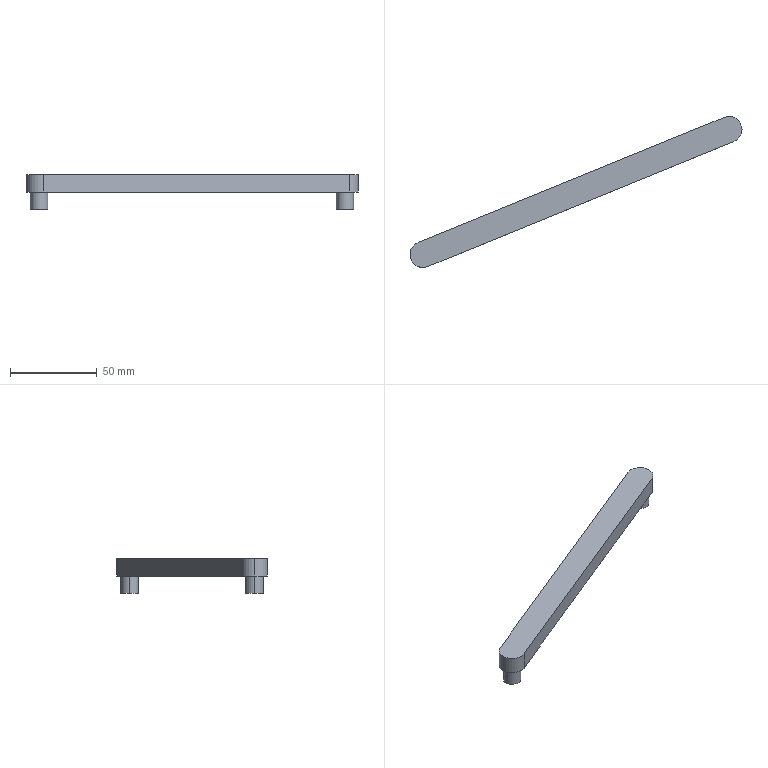Component | SolidWorks | CRocker-4 | 1 solid | 13 faces | box 190.9 x 86.82 x 20 mm | volume 31838 mm3 | cylinder 7 | plane 6 | commonest cylinder face diameters 10 x4 15 x3
build123d program:
from build123d import *

# Parameters (mm, degrees)
BOSS_EXTRUDE1_DEPTH = 10
SKETCH1_3_2_R       = 5
BOSS_EXTRUDE2_DEPTH = 10


with BuildPart() as part:
    # Sketch1_3 → Boss-Extrude1 (new body)
    with BuildSketch(Plane.XY):
        with BuildLine():
            Line((-32.504, 30.358), (-210.873, -35.098))
            ThreePointArc((-210.873, -35.098), (-220.498, -30.641), (-216.041, -21.016))
            Line((-216.041, -21.016), (-37.672, 44.44))
            ThreePointArc((-37.672, 44.44), (-28.047, 39.983), (-32.504, 30.358))
        make_face()
    extrude(amount=BOSS_EXTRUDE1_DEPTH)

    # Sketch1_3 2 → Boss-Extrude2 (add)
    with BuildSketch(Plane.XY):
        with Locations((-35.088, 37.399)):
            Circle(SKETCH1_3_2_R)
        with Locations((-213.457, -28.057)):
            Circle(SKETCH1_3_2_R)
    extrude(amount=-BOSS_EXTRUDE2_DEPTH)


solid = part.part

# Placed as in the assembly
solid = solid.moved(Location((215.701, -17.342, 137.182), (0, 0, 2.058)))
STEP:
#1=COLOUR_RGB('',0.7922,0.8196,0.9333);
#2=FILL_AREA_STYLE_COLOUR('',#1);
#3=FILL_AREA_STYLE('',(#2));
#4=SURFACE_STYLE_FILL_AREA(#3);
#5=SURFACE_SIDE_STYLE('',(#4));
#6=SURFACE_STYLE_USAGE(.BOTH.,#5);
#7=PRESENTATION_STYLE_ASSIGNMENT((#6));
#8=CARTESIAN_POINT('',(0.3301,-2.081,5.007));
#9=VERTEX_POINT('',#8);
#10=CARTESIAN_POINT('',(-0.06331,-2.095,5.007));
#11=VERTEX_POINT('',#10);
#12=CARTESIAN_POINT('',(0.1334,-2.088,5.007));
#13=DIRECTION('',(0.,0.,1.));
#14=DIRECTION('',(0.9994,0.0359,0.));
#15=AXIS2_PLACEMENT_3D('',#12,#13,#14);
#16=CIRCLE('',#15,0.1969);
#17=EDGE_CURVE('',#9,#11,#16,.T.);
#18=ORIENTED_EDGE('',*,*,#17,.T.);
#19=CARTESIAN_POINT('',(-0.06331,-2.095,5.401));
#20=VERTEX_POINT('',#19);
#21=CARTESIAN_POINT('',(-0.06331,-2.095,5.007));
#22=DIRECTION('',(0.,0.,1.));
#23=VECTOR('',#22,39.37);
#24=LINE('',#21,#23);
#25=EDGE_CURVE('',#11,#20,#24,.T.);
#26=ORIENTED_EDGE('',*,*,#25,.T.);
#27=CARTESIAN_POINT('',(0.3301,-2.081,5.401));
#28=VERTEX_POINT('',#27);
#29=CARTESIAN_POINT('',(0.1334,-2.088,5.401));
#30=DIRECTION('',(0.,0.,1.));
#31=DIRECTION('',(0.9994,0.0359,0.));
#32=AXIS2_PLACEMENT_3D('',#29,#30,#31);
#33=CIRCLE('',#32,0.1969);
#34=EDGE_CURVE('',#28,#20,#33,.T.);
#35=ORIENTED_EDGE('',*,*,#34,.F.);
#36=CARTESIAN_POINT('',(0.3301,-2.081,5.007));
#37=DIRECTION('',(0.,0.,1.));
#38=VECTOR('',#37,39.37);
#39=LINE('',#36,#38);
#40=EDGE_CURVE('',#9,#28,#39,.T.);
#41=ORIENTED_EDGE('',*,*,#40,.F.);
#42=EDGE_LOOP('',(#18,#26,#35,#41));
#43=FACE_OUTER_BOUND('',#42,.T.);
#44=CARTESIAN_POINT('',(0.1334,-2.088,5.007));
#45=DIRECTION('',(0.,0.,1.));
#46=DIRECTION('',(0.9994,0.0359,0.));
#47=AXIS2_PLACEMENT_3D('',#44,#45,#46);
#48=CYLINDRICAL_SURFACE('',#47,0.1969);
#49=ADVANCED_FACE('',(#43),#48,.T.);
#50=CARTESIAN_POINT('',(7.255,0.7462,5.007));
#51=VERTEX_POINT('',#50);
#52=CARTESIAN_POINT('',(6.862,0.732,5.007));
#53=VERTEX_POINT('',#52);
#54=CARTESIAN_POINT('',(7.059,0.7391,5.007));
#55=DIRECTION('',(0.,0.,1.));
#56=DIRECTION('',(0.9994,0.0359,0.));
#57=AXIS2_PLACEMENT_3D('',#54,#55,#56);
#58=CIRCLE('',#57,0.1969);
#59=EDGE_CURVE('',#51,#53,#58,.T.);
#60=ORIENTED_EDGE('',*,*,#59,.T.);
#61=CARTESIAN_POINT('',(6.862,0.732,5.401));
#62=VERTEX_POINT('',#61);
#63=CARTESIAN_POINT('',(6.862,0.732,5.007));
#64=DIRECTION('',(0.,0.,1.));
#65=VECTOR('',#64,39.37);
#66=LINE('',#63,#65);
#67=EDGE_CURVE('',#53,#62,#66,.T.);
#68=ORIENTED_EDGE('',*,*,#67,.T.);
#69=CARTESIAN_POINT('',(7.255,0.7462,5.401));
#70=VERTEX_POINT('',#69);
#71=CARTESIAN_POINT('',(7.059,0.7391,5.401));
#72=DIRECTION('',(0.,0.,1.));
#73=DIRECTION('',(0.9994,0.0359,0.));
#74=AXIS2_PLACEMENT_3D('',#71,#72,#73);
#75=CIRCLE('',#74,0.1969);
#76=EDGE_CURVE('',#70,#62,#75,.T.);
#77=ORIENTED_EDGE('',*,*,#76,.F.);
#78=CARTESIAN_POINT('',(7.255,0.7462,5.007));
#79=DIRECTION('',(0.,0.,1.));
#80=VECTOR('',#79,39.37);
#81=LINE('',#78,#80);
#82=EDGE_CURVE('',#51,#70,#81,.T.);
#83=ORIENTED_EDGE('',*,*,#82,.F.);
#84=EDGE_LOOP('',(#60,#68,#77,#83));
#85=FACE_OUTER_BOUND('',#84,.T.);
#86=CARTESIAN_POINT('',(7.059,0.7391,5.007));
#87=DIRECTION('',(0.,0.,1.));
#88=DIRECTION('',(0.9994,0.0359,0.));
#89=AXIS2_PLACEMENT_3D('',#86,#87,#88);
#90=CYLINDRICAL_SURFACE('',#89,0.1969);
#91=ADVANCED_FACE('',(#85),#90,.T.);
#92=CARTESIAN_POINT('',(-0.1617,-2.099,5.795));
#93=VERTEX_POINT('',#92);
#94=CARTESIAN_POINT('',(0.245,-2.362,5.795));
#95=VERTEX_POINT('',#94);
#96=CARTESIAN_POINT('',(0.1334,-2.088,5.795));
#97=DIRECTION('',(0.,0.,1.));
#98=DIRECTION('',(0.9994,0.0359,0.));
#99=AXIS2_PLACEMENT_3D('',#96,#97,#98);
#100=CIRCLE('',#99,0.2953);
#101=EDGE_CURVE('',#93,#95,#100,.T.);
#102=ORIENTED_EDGE('',*,*,#101,.F.);
#103=CARTESIAN_POINT('',(-0.1617,-2.099,5.401));
#104=VERTEX_POINT('',#103);
#105=CARTESIAN_POINT('',(-0.1617,-2.099,5.795));
#106=DIRECTION('',(-0.,-0.,-1.));
#107=VECTOR('',#106,39.37);
#108=LINE('',#105,#107);
#109=EDGE_CURVE('',#93,#104,#108,.T.);
#110=ORIENTED_EDGE('',*,*,#109,.T.);
#111=CARTESIAN_POINT('',(0.245,-2.362,5.401));
#112=VERTEX_POINT('',#111);
#113=CARTESIAN_POINT('',(0.1334,-2.088,5.401));
#114=DIRECTION('',(0.,0.,1.));
#115=DIRECTION('',(0.9994,0.0359,0.));
#116=AXIS2_PLACEMENT_3D('',#113,#114,#115);
#117=CIRCLE('',#116,0.2953);
#118=EDGE_CURVE('',#104,#112,#117,.T.);
#119=ORIENTED_EDGE('',*,*,#118,.T.);
#120=CARTESIAN_POINT('',(0.245,-2.362,5.795));
#121=DIRECTION('',(-0.,-0.,-1.));
#122=VECTOR('',#121,39.37);
#123=LINE('',#120,#122);
#124=EDGE_CURVE('',#95,#112,#123,.T.);
#125=ORIENTED_EDGE('',*,*,#124,.F.);
#126=EDGE_LOOP('',(#102,#110,#119,#125));
#127=FACE_OUTER_BOUND('',#126,.T.);
#128=CARTESIAN_POINT('',(0.1334,-2.088,5.795));
#129=DIRECTION('',(-0.,-0.,-1.));
#130=DIRECTION('',(-0.9994,-0.0359,0.));
#131=AXIS2_PLACEMENT_3D('',#128,#129,#130);
#132=CYLINDRICAL_SURFACE('',#131,0.2953);
#133=ADVANCED_FACE('',(#127),#132,.T.);
#134=CARTESIAN_POINT('',(6.947,1.012,5.795));
#135=VERTEX_POINT('',#134);
#136=CARTESIAN_POINT('',(0.0218,-1.815,5.795));
#137=VERTEX_POINT('',#136);
#138=CARTESIAN_POINT('',(7.678,1.311,5.795));
#139=DIRECTION('',(-0.9258,-0.378,0.));
#140=VECTOR('',#139,39.37);
#141=LINE('',#138,#140);
#142=EDGE_CURVE('',#135,#137,#141,.T.);
#143=ORIENTED_EDGE('',*,*,#142,.T.);
#144=CARTESIAN_POINT('',(0.1334,-2.088,5.795));
#145=DIRECTION('',(0.,0.,1.));
#146=DIRECTION('',(0.9994,0.0359,0.));
#147=AXIS2_PLACEMENT_3D('',#144,#145,#146);
#148=CIRCLE('',#147,0.2953);
#149=EDGE_CURVE('',#137,#93,#148,.T.);
#150=ORIENTED_EDGE('',*,*,#149,.T.);
#151=ORIENTED_EDGE('',*,*,#101,.T.);
#152=CARTESIAN_POINT('',(7.17,0.4657,5.795));
#153=VERTEX_POINT('',#152);
#154=CARTESIAN_POINT('',(7.901,0.7642,5.795));
#155=DIRECTION('',(-0.9258,-0.378,0.));
#156=VECTOR('',#155,39.37);
#157=LINE('',#154,#156);
#158=EDGE_CURVE('',#153,#95,#157,.T.);
#159=ORIENTED_EDGE('',*,*,#158,.F.);
#160=CARTESIAN_POINT('',(7.059,0.7391,5.795));
#161=DIRECTION('',(0.,0.,1.));
#162=DIRECTION('',(0.9994,0.0359,0.));
#163=AXIS2_PLACEMENT_3D('',#160,#161,#162);
#164=CIRCLE('',#163,0.2953);
#165=EDGE_CURVE('',#153,#135,#164,.T.);
#166=ORIENTED_EDGE('',*,*,#165,.T.);
#167=EDGE_LOOP('',(#143,#150,#151,#159,#166));
#168=FACE_OUTER_BOUND('',#167,.T.);
#169=CARTESIAN_POINT('',(8.492,-0.6828,5.795));
#170=DIRECTION('',(0.,0.,1.));
#171=DIRECTION('',(0.9994,0.0359,-0.));
#172=AXIS2_PLACEMENT_3D('',#169,#170,#171);
#173=PLANE('',#172);
#174=ADVANCED_FACE('',(#168),#173,.T.);
#175=ORIENTED_EDGE('',*,*,#34,.T.);
#176=CARTESIAN_POINT('',(0.1334,-2.088,5.401));
#177=DIRECTION('',(0.,0.,1.));
#178=DIRECTION('',(0.9994,0.0359,0.));
#179=AXIS2_PLACEMENT_3D('',#176,#177,#178);
#180=CIRCLE('',#179,0.1969);
#181=EDGE_CURVE('',#20,#28,#180,.T.);
#182=ORIENTED_EDGE('',*,*,#181,.T.);
#183=EDGE_LOOP('',(#175,#182));
#184=FACE_BOUND('',#183,.T.);
#185=ORIENTED_EDGE('',*,*,#76,.T.);
#186=CARTESIAN_POINT('',(7.059,0.7391,5.401));
#187=DIRECTION('',(0.,0.,1.));
#188=DIRECTION('',(0.9994,0.0359,0.));
#189=AXIS2_PLACEMENT_3D('',#186,#187,#188);
#190=CIRCLE('',#189,0.1969);
#191=EDGE_CURVE('',#62,#70,#190,.T.);
#192=ORIENTED_EDGE('',*,*,#191,.T.);
#193=EDGE_LOOP('',(#185,#192));
#194=FACE_BOUND('',#193,.T.);
#195=CARTESIAN_POINT('',(6.947,1.012,5.401));
#196=VERTEX_POINT('',#195);
#197=CARTESIAN_POINT('',(0.0218,-1.815,5.401));
#198=VERTEX_POINT('',#197);
#199=CARTESIAN_POINT('',(7.678,1.311,5.401));
#200=DIRECTION('',(-0.9258,-0.378,0.));
#201=VECTOR('',#200,39.37);
#202=LINE('',#199,#201);
#203=EDGE_CURVE('',#196,#198,#202,.T.);
#204=ORIENTED_EDGE('',*,*,#203,.F.);
#205=CARTESIAN_POINT('',(7.17,0.4657,5.401));
#206=VERTEX_POINT('',#205);
#207=CARTESIAN_POINT('',(7.059,0.7391,5.401));
#208=DIRECTION('',(0.,0.,1.));
#209=DIRECTION('',(0.9994,0.0359,0.));
#210=AXIS2_PLACEMENT_3D('',#207,#208,#209);
#211=CIRCLE('',#210,0.2953);
#212=EDGE_CURVE('',#206,#196,#211,.T.);
#213=ORIENTED_EDGE('',*,*,#212,.F.);
#214=CARTESIAN_POINT('',(7.901,0.7642,5.401));
#215=DIRECTION('',(-0.9258,-0.378,0.));
#216=VECTOR('',#215,39.37);
#217=LINE('',#214,#216);
#218=EDGE_CURVE('',#206,#112,#217,.T.);
#219=ORIENTED_EDGE('',*,*,#218,.T.);
#220=ORIENTED_EDGE('',*,*,#118,.F.);
#221=CARTESIAN_POINT('',(0.1334,-2.088,5.401));
#222=DIRECTION('',(0.,0.,1.));
#223=DIRECTION('',(0.9994,0.0359,0.));
#224=AXIS2_PLACEMENT_3D('',#221,#222,#223);
#225=CIRCLE('',#224,0.2953);
#226=EDGE_CURVE('',#198,#104,#225,.T.);
#227=ORIENTED_EDGE('',*,*,#226,.F.);
#228=EDGE_LOOP('',(#204,#213,#219,#220,#227));
#229=FACE_OUTER_BOUND('',#228,.T.);
#230=CARTESIAN_POINT('',(8.492,-0.6828,5.401));
#231=DIRECTION('',(0.,0.,1.));
#232=DIRECTION('',(0.9994,0.0359,-0.));
#233=AXIS2_PLACEMENT_3D('',#230,#231,#232);
#234=PLANE('',#233);
#235=ADVANCED_FACE('',(#184,#194,#229),#234,.F.);
#236=ORIENTED_EDGE('',*,*,#109,.F.);
#237=ORIENTED_EDGE('',*,*,#149,.F.);
#238=CARTESIAN_POINT('',(0.0218,-1.815,5.795));
#239=DIRECTION('',(-0.,-0.,-1.));
#240=VECTOR('',#239,39.37);
#241=LINE('',#238,#240);
#242=EDGE_CURVE('',#137,#198,#241,.T.);
#243=ORIENTED_EDGE('',*,*,#242,.T.);
#244=ORIENTED_EDGE('',*,*,#226,.T.);
#245=EDGE_LOOP('',(#236,#237,#243,#244));
#246=FACE_OUTER_BOUND('',#245,.T.);
#247=CARTESIAN_POINT('',(0.1334,-2.088,5.795));
#248=DIRECTION('',(-0.,-0.,-1.));
#249=DIRECTION('',(-0.9994,-0.0359,0.));
#250=AXIS2_PLACEMENT_3D('',#247,#248,#249);
#251=CYLINDRICAL_SURFACE('',#250,0.2953);
#252=ADVANCED_FACE('',(#246),#251,.T.);
#253=ORIENTED_EDGE('',*,*,#218,.F.);
#254=CARTESIAN_POINT('',(7.17,0.4657,5.795));
#255=DIRECTION('',(-0.,-0.,-1.));
#256=VECTOR('',#255,39.37);
#257=LINE('',#254,#256);
#258=EDGE_CURVE('',#153,#206,#257,.T.);
#259=ORIENTED_EDGE('',*,*,#258,.F.);
#260=ORIENTED_EDGE('',*,*,#158,.T.);
#261=ORIENTED_EDGE('',*,*,#124,.T.);
#262=EDGE_LOOP('',(#253,#259,#260,#261));
#263=FACE_OUTER_BOUND('',#262,.T.);
#264=CARTESIAN_POINT('',(7.901,0.7642,5.795));
#265=DIRECTION('',(0.378,-0.9258,-0.));
#266=DIRECTION('',(0.9258,0.378,-0.));
#267=AXIS2_PLACEMENT_3D('',#264,#265,#266);
#268=PLANE('',#267);
#269=ADVANCED_FACE('',(#263),#268,.T.);
#270=ORIENTED_EDGE('',*,*,#212,.T.);
#271=CARTESIAN_POINT('',(6.947,1.012,5.795));
#272=DIRECTION('',(-0.,-0.,-1.));
#273=VECTOR('',#272,39.37);
#274=LINE('',#271,#273);
#275=EDGE_CURVE('',#135,#196,#274,.T.);
#276=ORIENTED_EDGE('',*,*,#275,.F.);
#277=ORIENTED_EDGE('',*,*,#165,.F.);
#278=ORIENTED_EDGE('',*,*,#258,.T.);
#279=EDGE_LOOP('',(#270,#276,#277,#278));
#280=FACE_OUTER_BOUND('',#279,.T.);
#281=CARTESIAN_POINT('',(7.059,0.7391,5.795));
#282=DIRECTION('',(-0.,-0.,-1.));
#283=DIRECTION('',(-0.9994,-0.0359,0.));
#284=AXIS2_PLACEMENT_3D('',#281,#282,#283);
#285=CYLINDRICAL_SURFACE('',#284,0.2953);
#286=ADVANCED_FACE('',(#280),#285,.T.);
#287=ORIENTED_EDGE('',*,*,#203,.T.);
#288=ORIENTED_EDGE('',*,*,#242,.F.);
#289=ORIENTED_EDGE('',*,*,#142,.F.);
#290=ORIENTED_EDGE('',*,*,#275,.T.);
#291=EDGE_LOOP('',(#287,#288,#289,#290));
#292=FACE_OUTER_BOUND('',#291,.T.);
#293=CARTESIAN_POINT('',(7.678,1.311,5.795));
#294=DIRECTION('',(0.378,-0.9258,-0.));
#295=DIRECTION('',(0.9258,0.378,-0.));
#296=AXIS2_PLACEMENT_3D('',#293,#294,#295);
#297=PLANE('',#296);
#298=ADVANCED_FACE('',(#292),#297,.F.);
#299=ORIENTED_EDGE('',*,*,#67,.F.);
#300=CARTESIAN_POINT('',(7.059,0.7391,5.007));
#301=DIRECTION('',(0.,0.,1.));
#302=DIRECTION('',(0.9994,0.0359,0.));
#303=AXIS2_PLACEMENT_3D('',#300,#301,#302);
#304=CIRCLE('',#303,0.1969);
#305=EDGE_CURVE('',#53,#51,#304,.T.);
#306=ORIENTED_EDGE('',*,*,#305,.T.);
#307=ORIENTED_EDGE('',*,*,#82,.T.);
#308=ORIENTED_EDGE('',*,*,#191,.F.);
#309=EDGE_LOOP('',(#299,#306,#307,#308));
#310=FACE_OUTER_BOUND('',#309,.T.);
#311=CARTESIAN_POINT('',(7.059,0.7391,5.007));
#312=DIRECTION('',(0.,0.,1.));
#313=DIRECTION('',(0.9994,0.0359,0.));
#314=AXIS2_PLACEMENT_3D('',#311,#312,#313);
#315=CYLINDRICAL_SURFACE('',#314,0.1969);
#316=ADVANCED_FACE('',(#310),#315,.T.);
#317=ORIENTED_EDGE('',*,*,#59,.F.);
#318=ORIENTED_EDGE('',*,*,#305,.F.);
#319=EDGE_LOOP('',(#317,#318));
#320=FACE_OUTER_BOUND('',#319,.T.);
#321=CARTESIAN_POINT('',(8.492,-0.6828,5.007));
#322=DIRECTION('',(0.,0.,1.));
#323=DIRECTION('',(0.9994,0.0359,-0.));
#324=AXIS2_PLACEMENT_3D('',#321,#322,#323);
#325=PLANE('',#324);
#326=ADVANCED_FACE('',(#320),#325,.F.);
#327=ORIENTED_EDGE('',*,*,#25,.F.);
#328=CARTESIAN_POINT('',(0.1334,-2.088,5.007));
#329=DIRECTION('',(0.,0.,1.));
#330=DIRECTION('',(0.9994,0.0359,0.));
#331=AXIS2_PLACEMENT_3D('',#328,#329,#330);
#332=CIRCLE('',#331,0.1969);
#333=EDGE_CURVE('',#11,#9,#332,.T.);
#334=ORIENTED_EDGE('',*,*,#333,.T.);
#335=ORIENTED_EDGE('',*,*,#40,.T.);
#336=ORIENTED_EDGE('',*,*,#181,.F.);
#337=EDGE_LOOP('',(#327,#334,#335,#336));
#338=FACE_OUTER_BOUND('',#337,.T.);
#339=CARTESIAN_POINT('',(0.1334,-2.088,5.007));
#340=DIRECTION('',(0.,0.,1.));
#341=DIRECTION('',(0.9994,0.0359,0.));
#342=AXIS2_PLACEMENT_3D('',#339,#340,#341);
#343=CYLINDRICAL_SURFACE('',#342,0.1969);
#344=ADVANCED_FACE('',(#338),#343,.T.);
#345=ORIENTED_EDGE('',*,*,#17,.F.);
#346=ORIENTED_EDGE('',*,*,#333,.F.);
#347=EDGE_LOOP('',(#345,#346));
#348=FACE_OUTER_BOUND('',#347,.T.);
#349=CARTESIAN_POINT('',(0.1334,-2.088,5.007));
#350=DIRECTION('',(0.,0.,1.));
#351=DIRECTION('',(0.9994,0.0359,-0.));
#352=AXIS2_PLACEMENT_3D('',#349,#350,#351);
#353=PLANE('',#352);
#354=ADVANCED_FACE('',(#348),#353,.F.);
#355=CLOSED_SHELL('',(#49,#91,#133,#174,#235,#252,#269,#286,#298,#316,#326,#344,#354));
#356=MANIFOLD_SOLID_BREP('',#355);
#357=STYLED_ITEM('',(#7),#356);
#358=PRESENTATION_LAYER_ASSIGNMENT('','',(#357));
#359=(LENGTH_UNIT()NAMED_UNIT(*)SI_UNIT($,.METRE.));
#360=LENGTH_MEASURE_WITH_UNIT(LENGTH_MEASURE(0.0254),#359);
#361=DIMENSIONAL_EXPONENTS(1.,0.,0.,0.,0.,0.,0.);
#362=(CONVERSION_BASED_UNIT('',#360)LENGTH_UNIT()NAMED_UNIT(#361));
#363=UNCERTAINTY_MEASURE_WITH_UNIT(LENGTH_MEASURE(0.00001),#362,'','');
#364=(NAMED_UNIT(*)PLANE_ANGLE_UNIT()SI_UNIT($,.RADIAN.));
#365=(NAMED_UNIT(*)SI_UNIT($,.STERADIAN.)SOLID_ANGLE_UNIT());
#366=(GEOMETRIC_REPRESENTATION_CONTEXT(3)GLOBAL_UNCERTAINTY_ASSIGNED_CONTEXT((#363))GLOBAL_UNIT_ASSIGNED_CONTEXT((#362,#364,#365))REPRESENTATION_CONTEXT('',''));
#367=MECHANICAL_DESIGN_GEOMETRIC_PRESENTATION_REPRESENTATION('',(#357),#366);
#368=CARTESIAN_POINT('',(0.,0.,0.));
#369=DIRECTION('',(0.,0.,1.));
#370=DIRECTION('',(1.,0.,0.));
#371=AXIS2_PLACEMENT_3D('',#368,#369,#370);
#372=(LENGTH_UNIT()NAMED_UNIT(*)SI_UNIT($,.METRE.));
#373=LENGTH_MEASURE_WITH_UNIT(LENGTH_MEASURE(0.0254),#372);
#374=DIMENSIONAL_EXPONENTS(1.,0.,0.,0.,0.,0.,0.);
#375=(CONVERSION_BASED_UNIT('',#373)LENGTH_UNIT()NAMED_UNIT(#374));
#376=UNCERTAINTY_MEASURE_WITH_UNIT(LENGTH_MEASURE(0.00001),#375,'','');
#377=(NAMED_UNIT(*)PLANE_ANGLE_UNIT()SI_UNIT($,.RADIAN.));
#378=(NAMED_UNIT(*)SI_UNIT($,.STERADIAN.)SOLID_ANGLE_UNIT());
#379=(GEOMETRIC_REPRESENTATION_CONTEXT(3)GLOBAL_UNCERTAINTY_ASSIGNED_CONTEXT((#376))GLOBAL_UNIT_ASSIGNED_CONTEXT((#375,#377,#378))REPRESENTATION_CONTEXT('',''));
#380=ADVANCED_BREP_SHAPE_REPRESENTATION('',(#356,#371),#379);